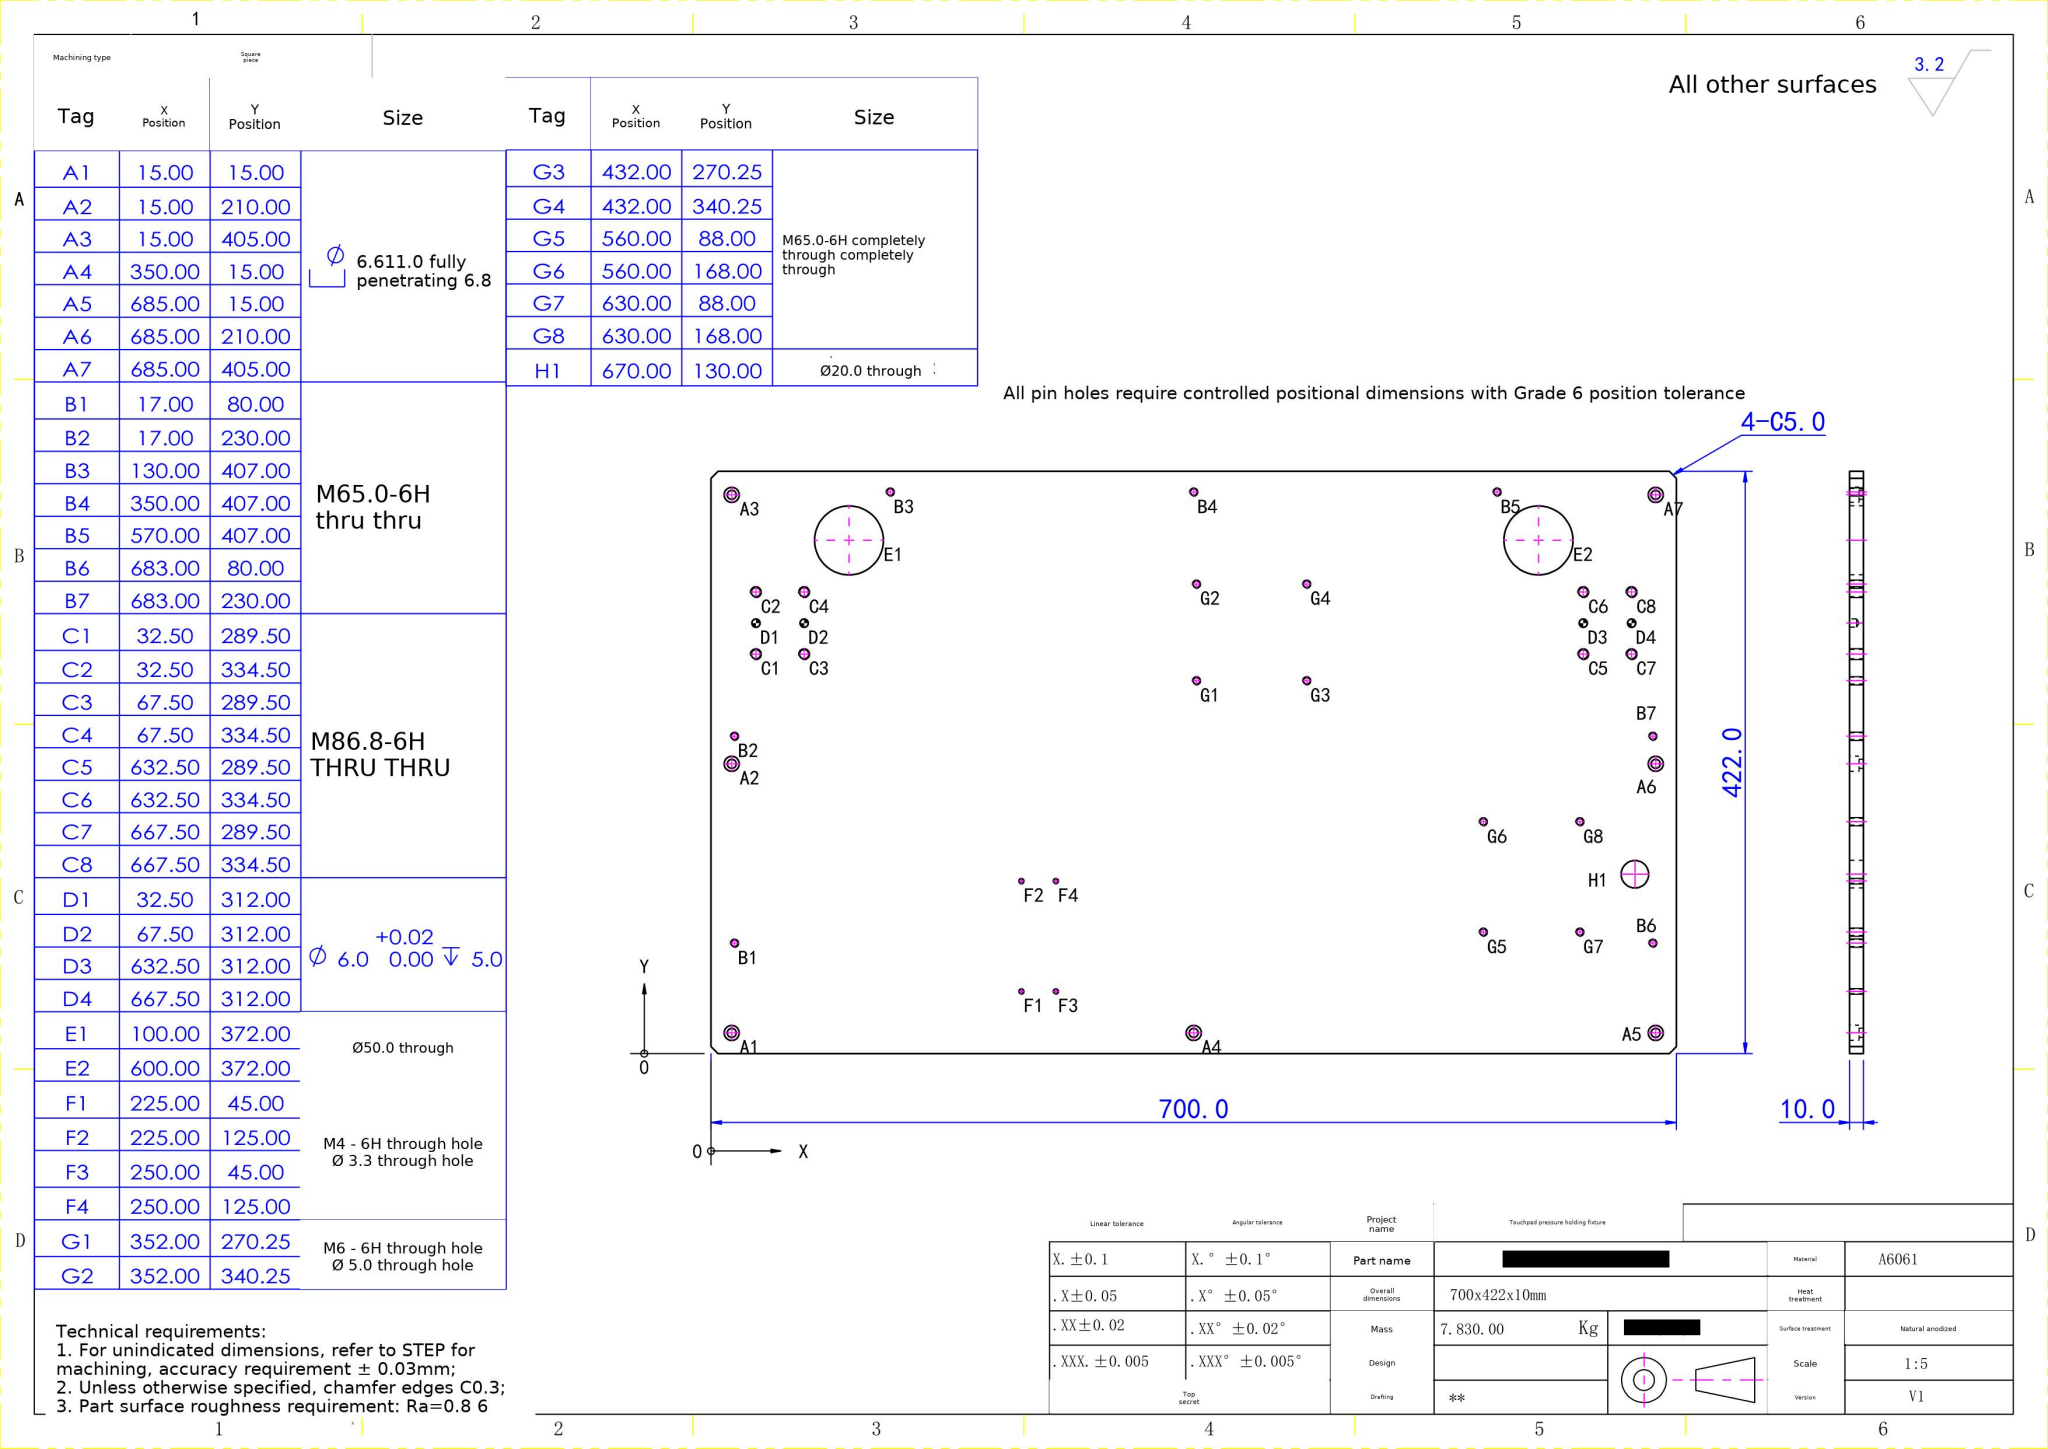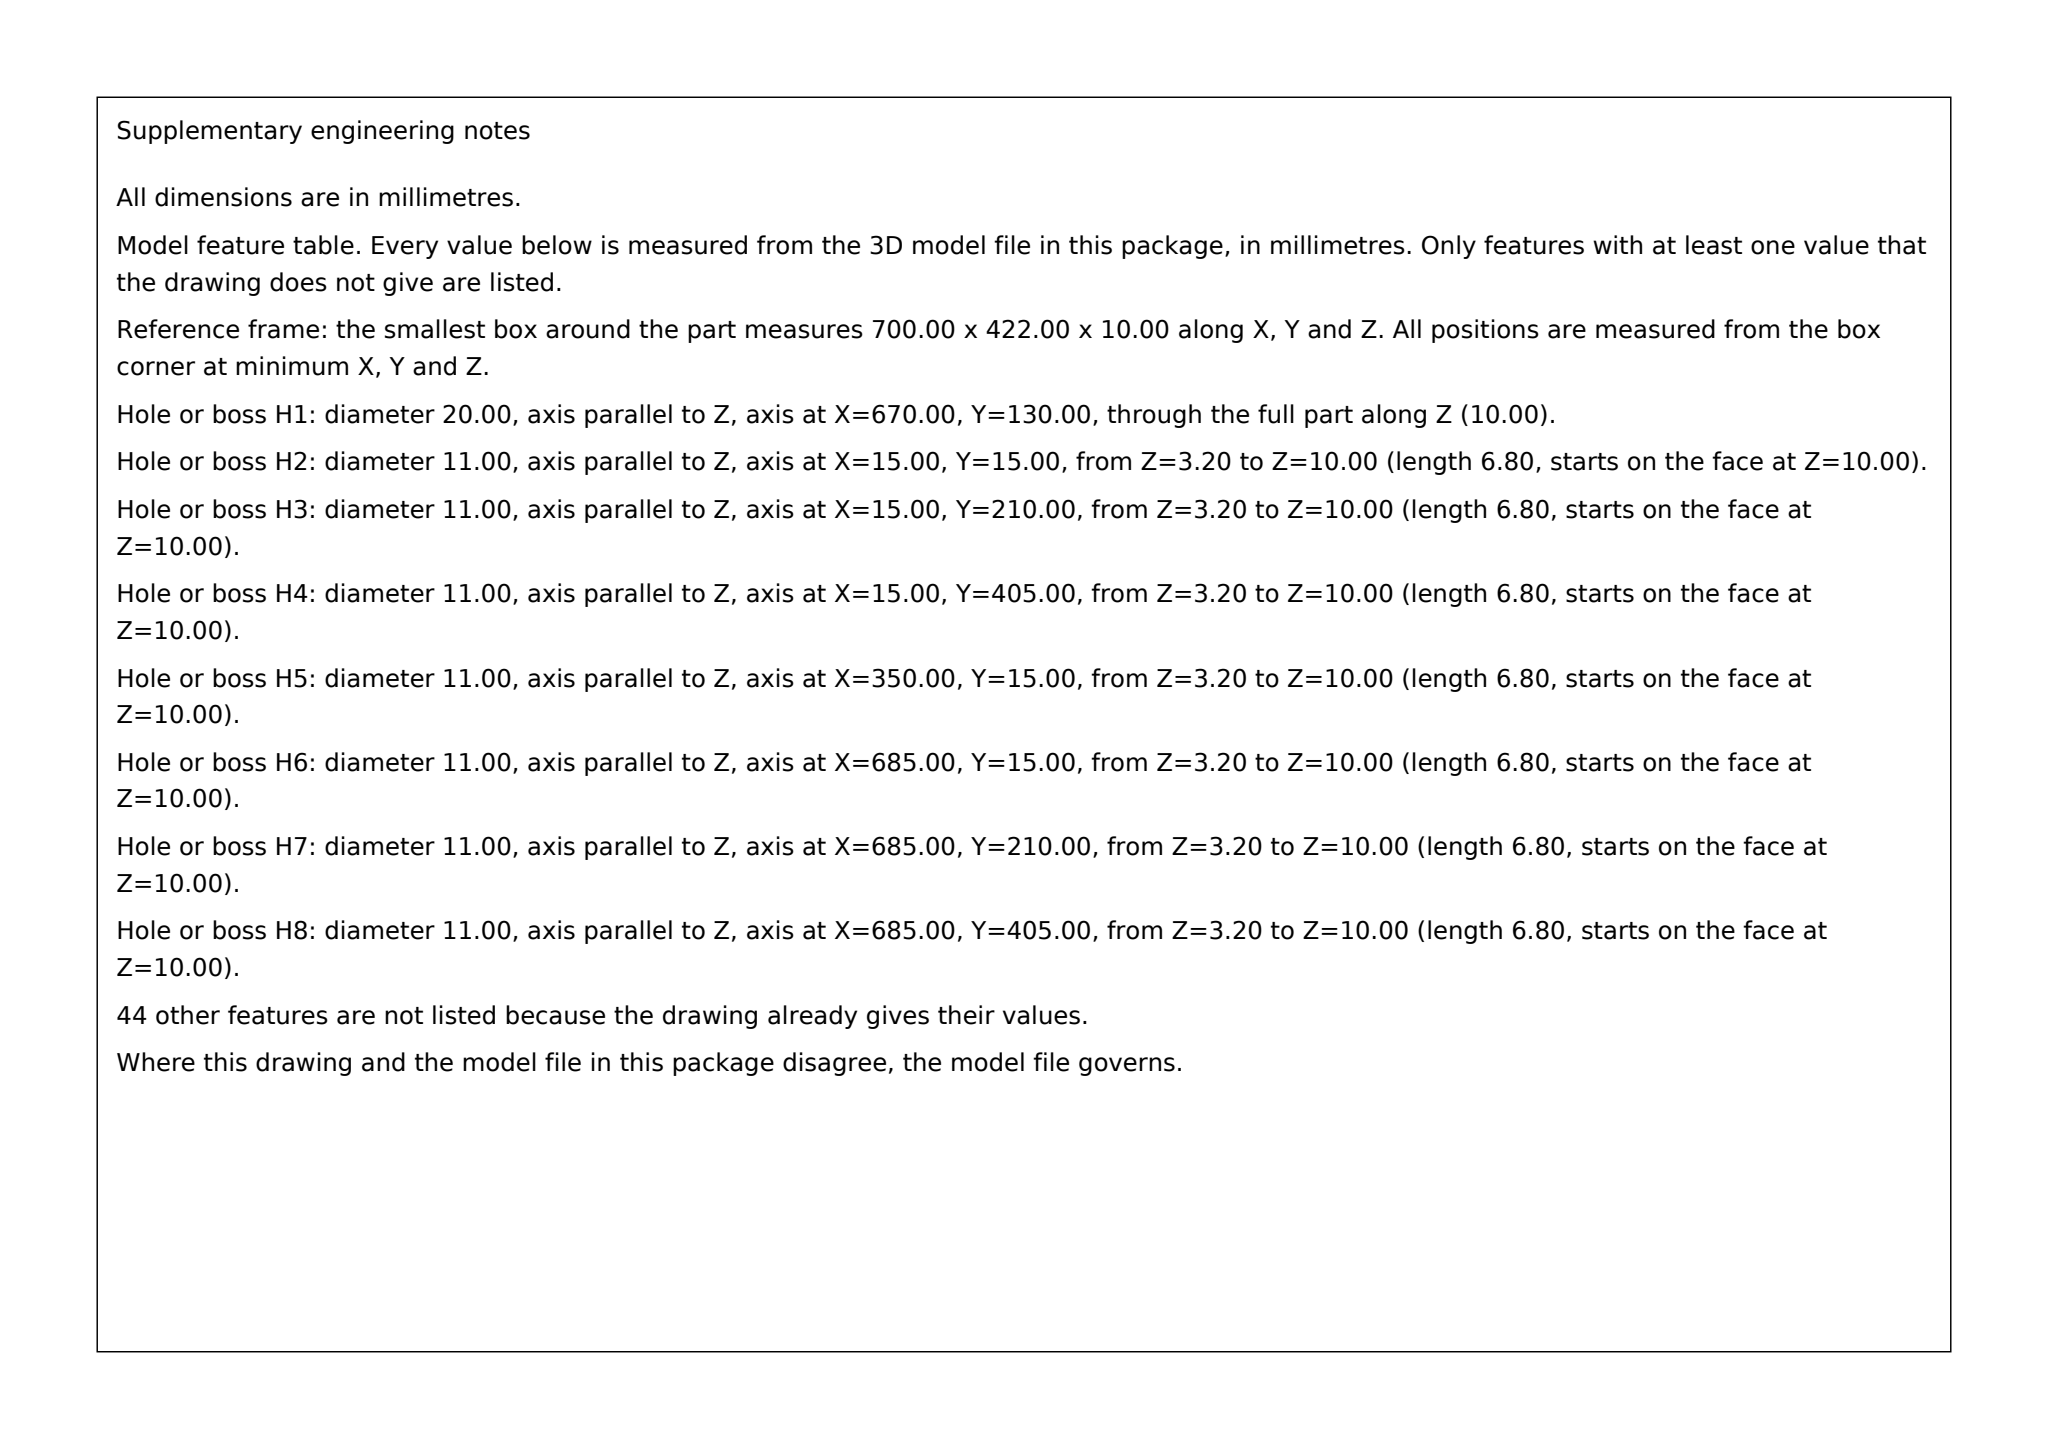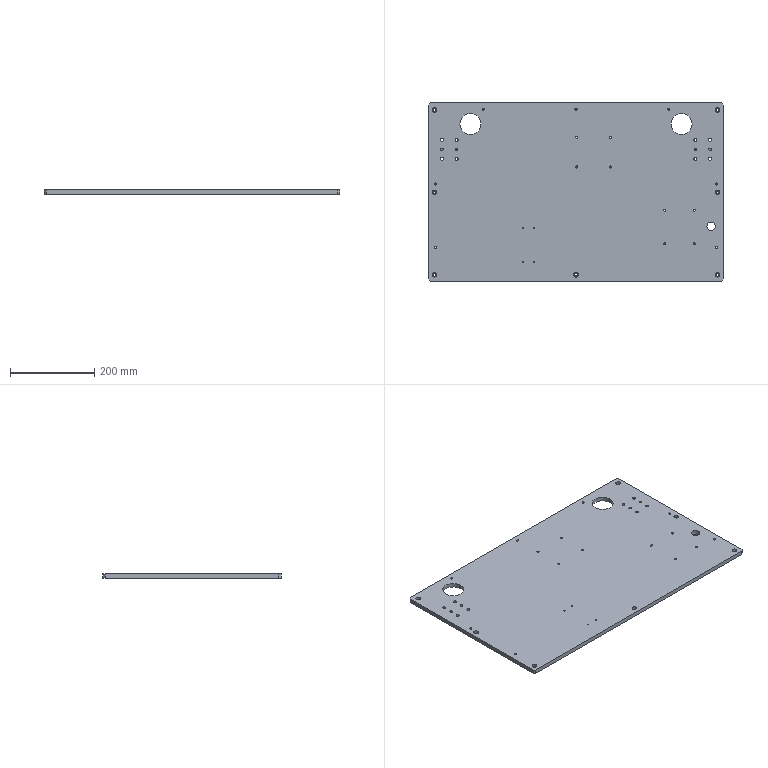Part | SolidWorks | mm | 1 solid | 121 faces | box 700 x 422 x 10 mm | volume 2898972 mm3 | cylinder 96 | plane 17 | cone 8 | commonest cylinder face diameters 5 x30 6.8 x16 11 x14 6.6 x14 3.3 x8 6 x8 50 x4 20 x2
build123d program:
from build123d import *

# Parameters (mm, degrees)
SKETCH1_W                                       = 700
SKETCH1_H                                       = 422
BOSS_EXTRUDE1_DEPTH                             = 10
SKETCH8_R                                       = 25
CUT_EXTRUDE2_DEPTH                              = 409.804
CHAMFER1_SIZE                                   = 5
M6_HEX_SOCKET_HEAD_CAP_SCREW_CBORE1_D           = 6.6
M6_HEX_SOCKET_HEAD_CAP_SCREW_CBORE1_CBORE_D     = 11
M6_HEX_SOCKET_HEAD_CAP_SCREW_CBORE1_CBORE_DEPTH = 6.8
M6_TAPPED_HOLE2_D                               = 5
M8_TAPPED_HOLE1_D                               = 6.8
F_6_0MM_DOWEL_HOLE1_D                           = 6
F_6_0MM_DOWEL_HOLE1_DEPTH                       = 5
F_6_0MM_DOWEL_HOLE1_TIP                         = 1.803
M4_TAPPED_HOLE3_D                               = 3.3
SKETCH44_R                                      = 10
CUT_EXTRUDE3_DEPTH                              = 409.804
M6_TAPPED_HOLE1_D                               = 5


with BuildPart() as part:
    # Sketch1 → Boss-Extrude1 (new body)
    with BuildSketch(Plane.XY):
        Rectangle(SKETCH1_W, SKETCH1_H)
    extrude(amount=BOSS_EXTRUDE1_DEPTH)

    # Sketch8 → Cut-Extrude2 (cut, through all)
    with BuildSketch(Plane.XY.offset(10)):
        with Locations((-250, 161)):
            Circle(SKETCH8_R)
        with Locations((250, 161)):
            Circle(SKETCH8_R)
    extrude(amount=-CUT_EXTRUDE2_DEPTH, mode=Mode.SUBTRACT)

    # Chamfer1
    chamfer1_edges = [part.edges().sort_by_distance(p)[0] for p in [
        (-350, 211, 5),
        (350, 211, 5),
        (350, -211, 5),
        (-350, -211, 5),
    ]]
    chamfer(chamfer1_edges, length=CHAMFER1_SIZE)

    # M6 Hex Socket Head Cap Screw CBORE1 (through all)
    with Locations(Plane.XY.offset(10)):
        with Locations((-335, -196), (335, -196), (0, -196), (-335, -1), (335, -1), (-335, 194), (335, 194)):
            CounterBoreHole(M6_HEX_SOCKET_HEAD_CAP_SCREW_CBORE1_D / 2, M6_HEX_SOCKET_HEAD_CAP_SCREW_CBORE1_CBORE_D / 2, M6_HEX_SOCKET_HEAD_CAP_SCREW_CBORE1_CBORE_DEPTH)

    # M6 Tapped Hole2 (through all)
    with Locations(Plane.XY.offset(10)):
        with Locations((-220, 196), (220, 196), (0, 196), (-333, 19), (-333, -131), (333, -131), (333, 19)):
            Hole(M6_TAPPED_HOLE2_D / 2)

    # M8 Tapped Hole1 (through all)
    with Locations(Plane.XY.offset(10)):
        with Locations((317.5, 78.5), (317.5, 123.5), (282.5, 123.5), (282.5, 78.5), (-282.5, 78.5), (-282.5, 123.5), (-317.5, 123.5), (-317.5, 78.5)):
            Hole(M8_TAPPED_HOLE1_D / 2)

    # 6.0mm Dowel Hole1
    with Locations(Plane.XY.offset(10)):
        with Locations((-317.5, 101), (-282.5, 101), (282.5, 101), (317.5, 101)):
            Hole(F_6_0MM_DOWEL_HOLE1_D / 2, depth=F_6_0MM_DOWEL_HOLE1_DEPTH)
            with Locations((0, 0, -(F_6_0MM_DOWEL_HOLE1_DEPTH + F_6_0MM_DOWEL_HOLE1_TIP / 2))):  # 118° drill point
                Cone(0, F_6_0MM_DOWEL_HOLE1_D / 2, F_6_0MM_DOWEL_HOLE1_TIP, mode=Mode.SUBTRACT)

    # M4 Tapped Hole3 (through all)
    with Locations(Plane.XY.offset(10)):
        with Locations((-125, -86), (-100, -86), (-125, -166), (-100, -166)):
            Hole(M4_TAPPED_HOLE3_D / 2)

    # Sketch44 → Cut-Extrude3 (cut, through all)
    with BuildSketch(Plane.XY.offset(10)):
        with Locations((320, -81)):
            Circle(SKETCH44_R)
    extrude(amount=-CUT_EXTRUDE3_DEPTH, mode=Mode.SUBTRACT)

    # M6 Tapped Hole1 (through all)
    with Locations(Plane.XY.offset(10)):
        with Locations((82, 129.248), (2, 129.248), (2, 59.248), (82, 59.248), (280, -43), (280, -123), (210, -43), (210, -123)):
            Hole(M6_TAPPED_HOLE1_D / 2)


solid = part.part